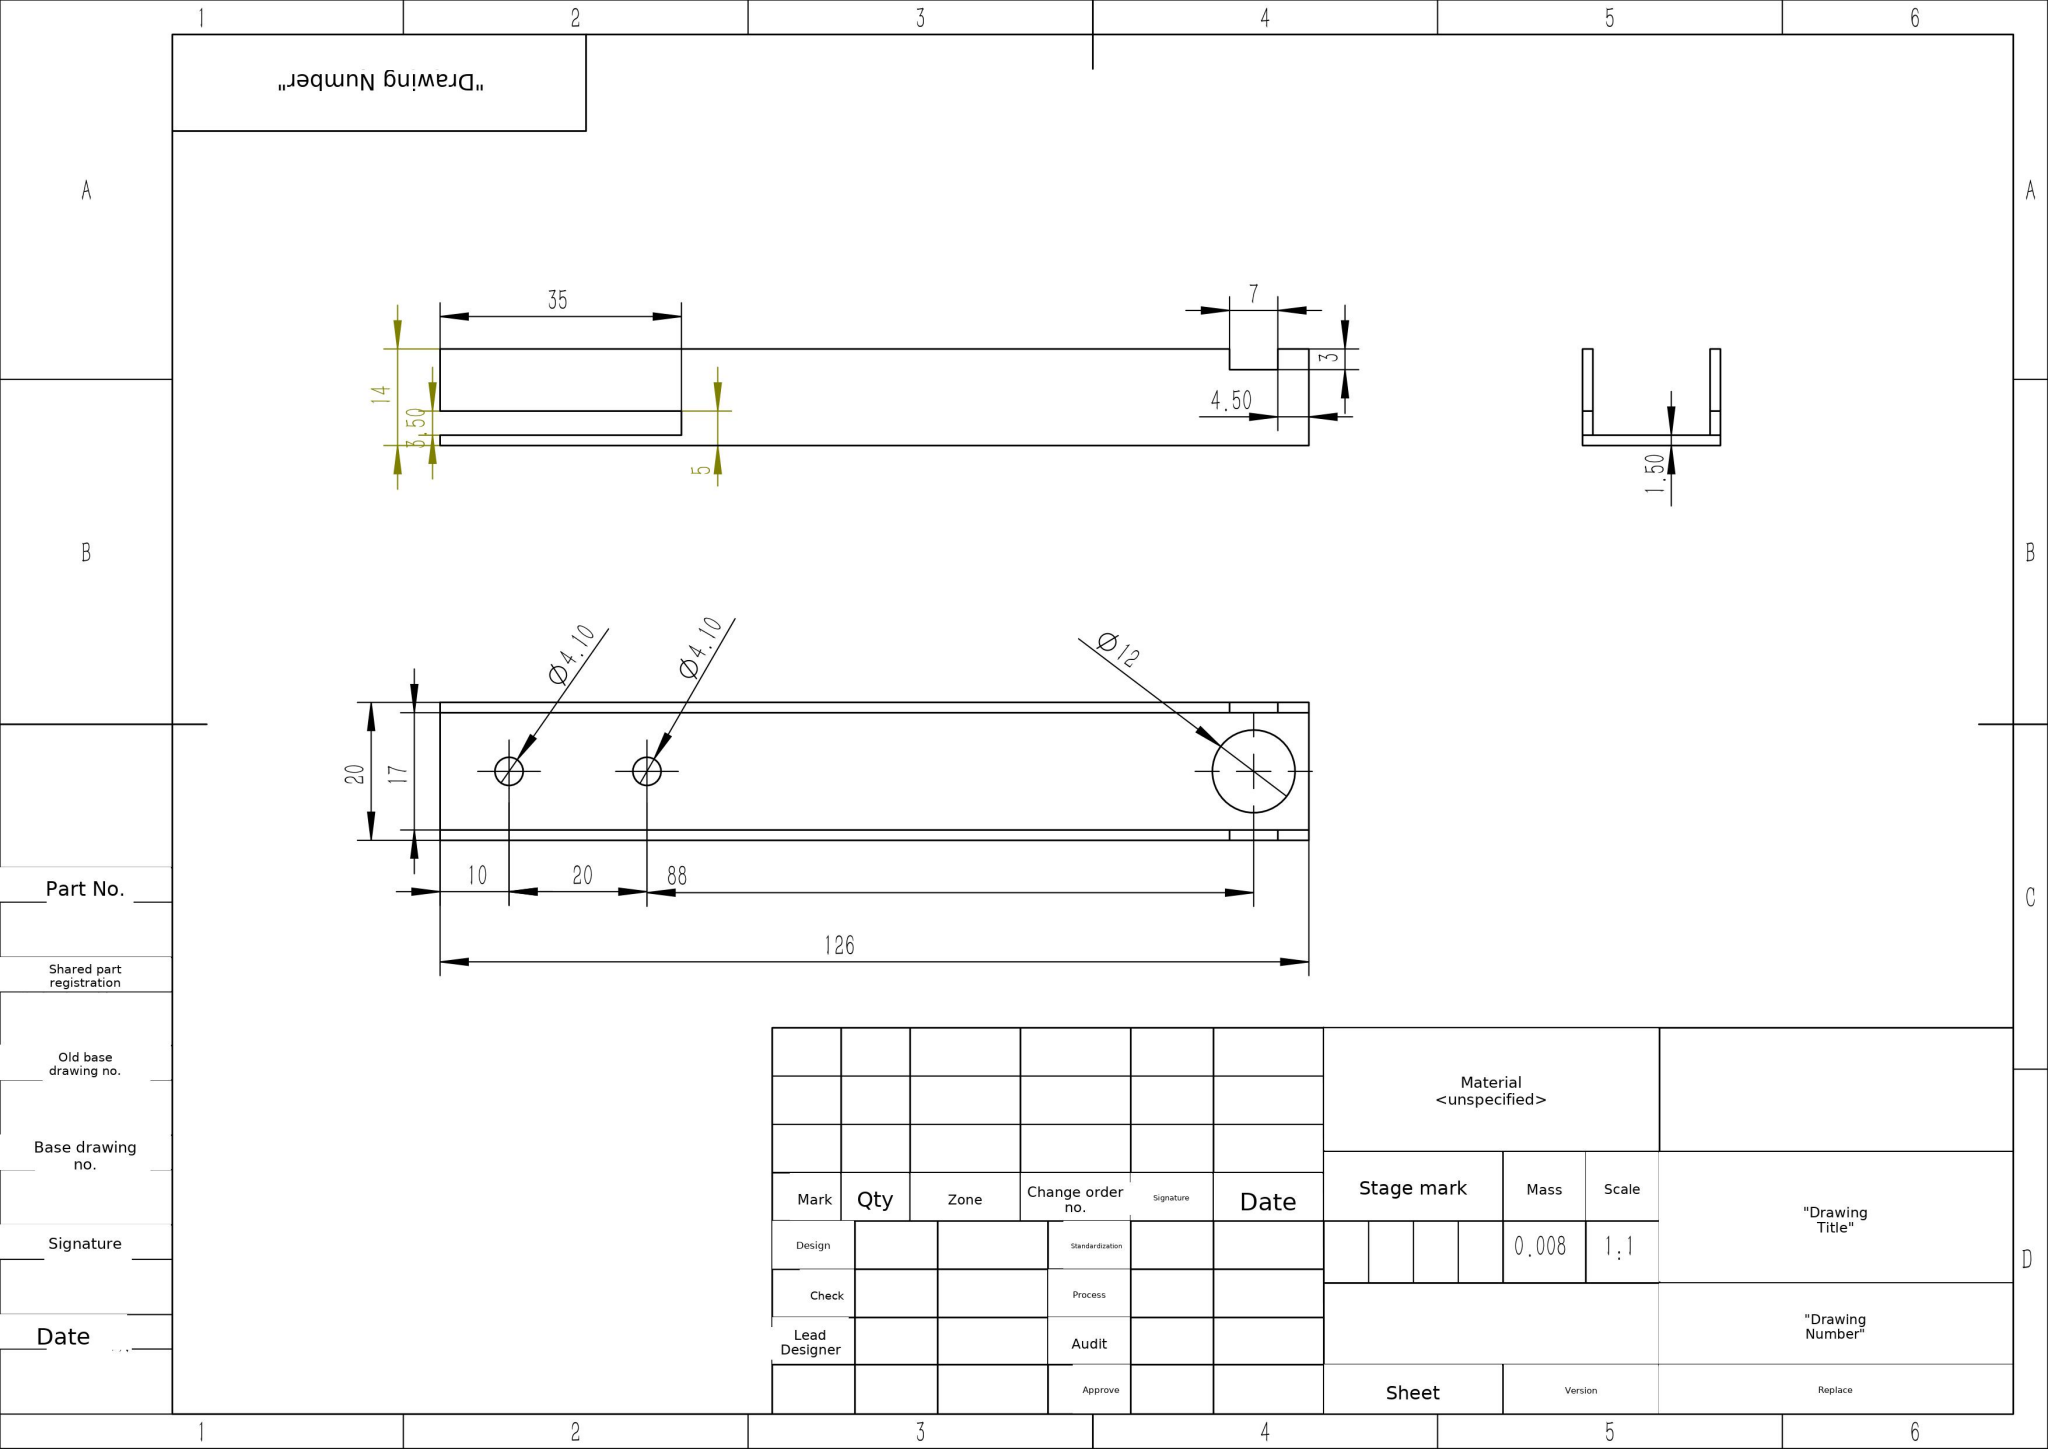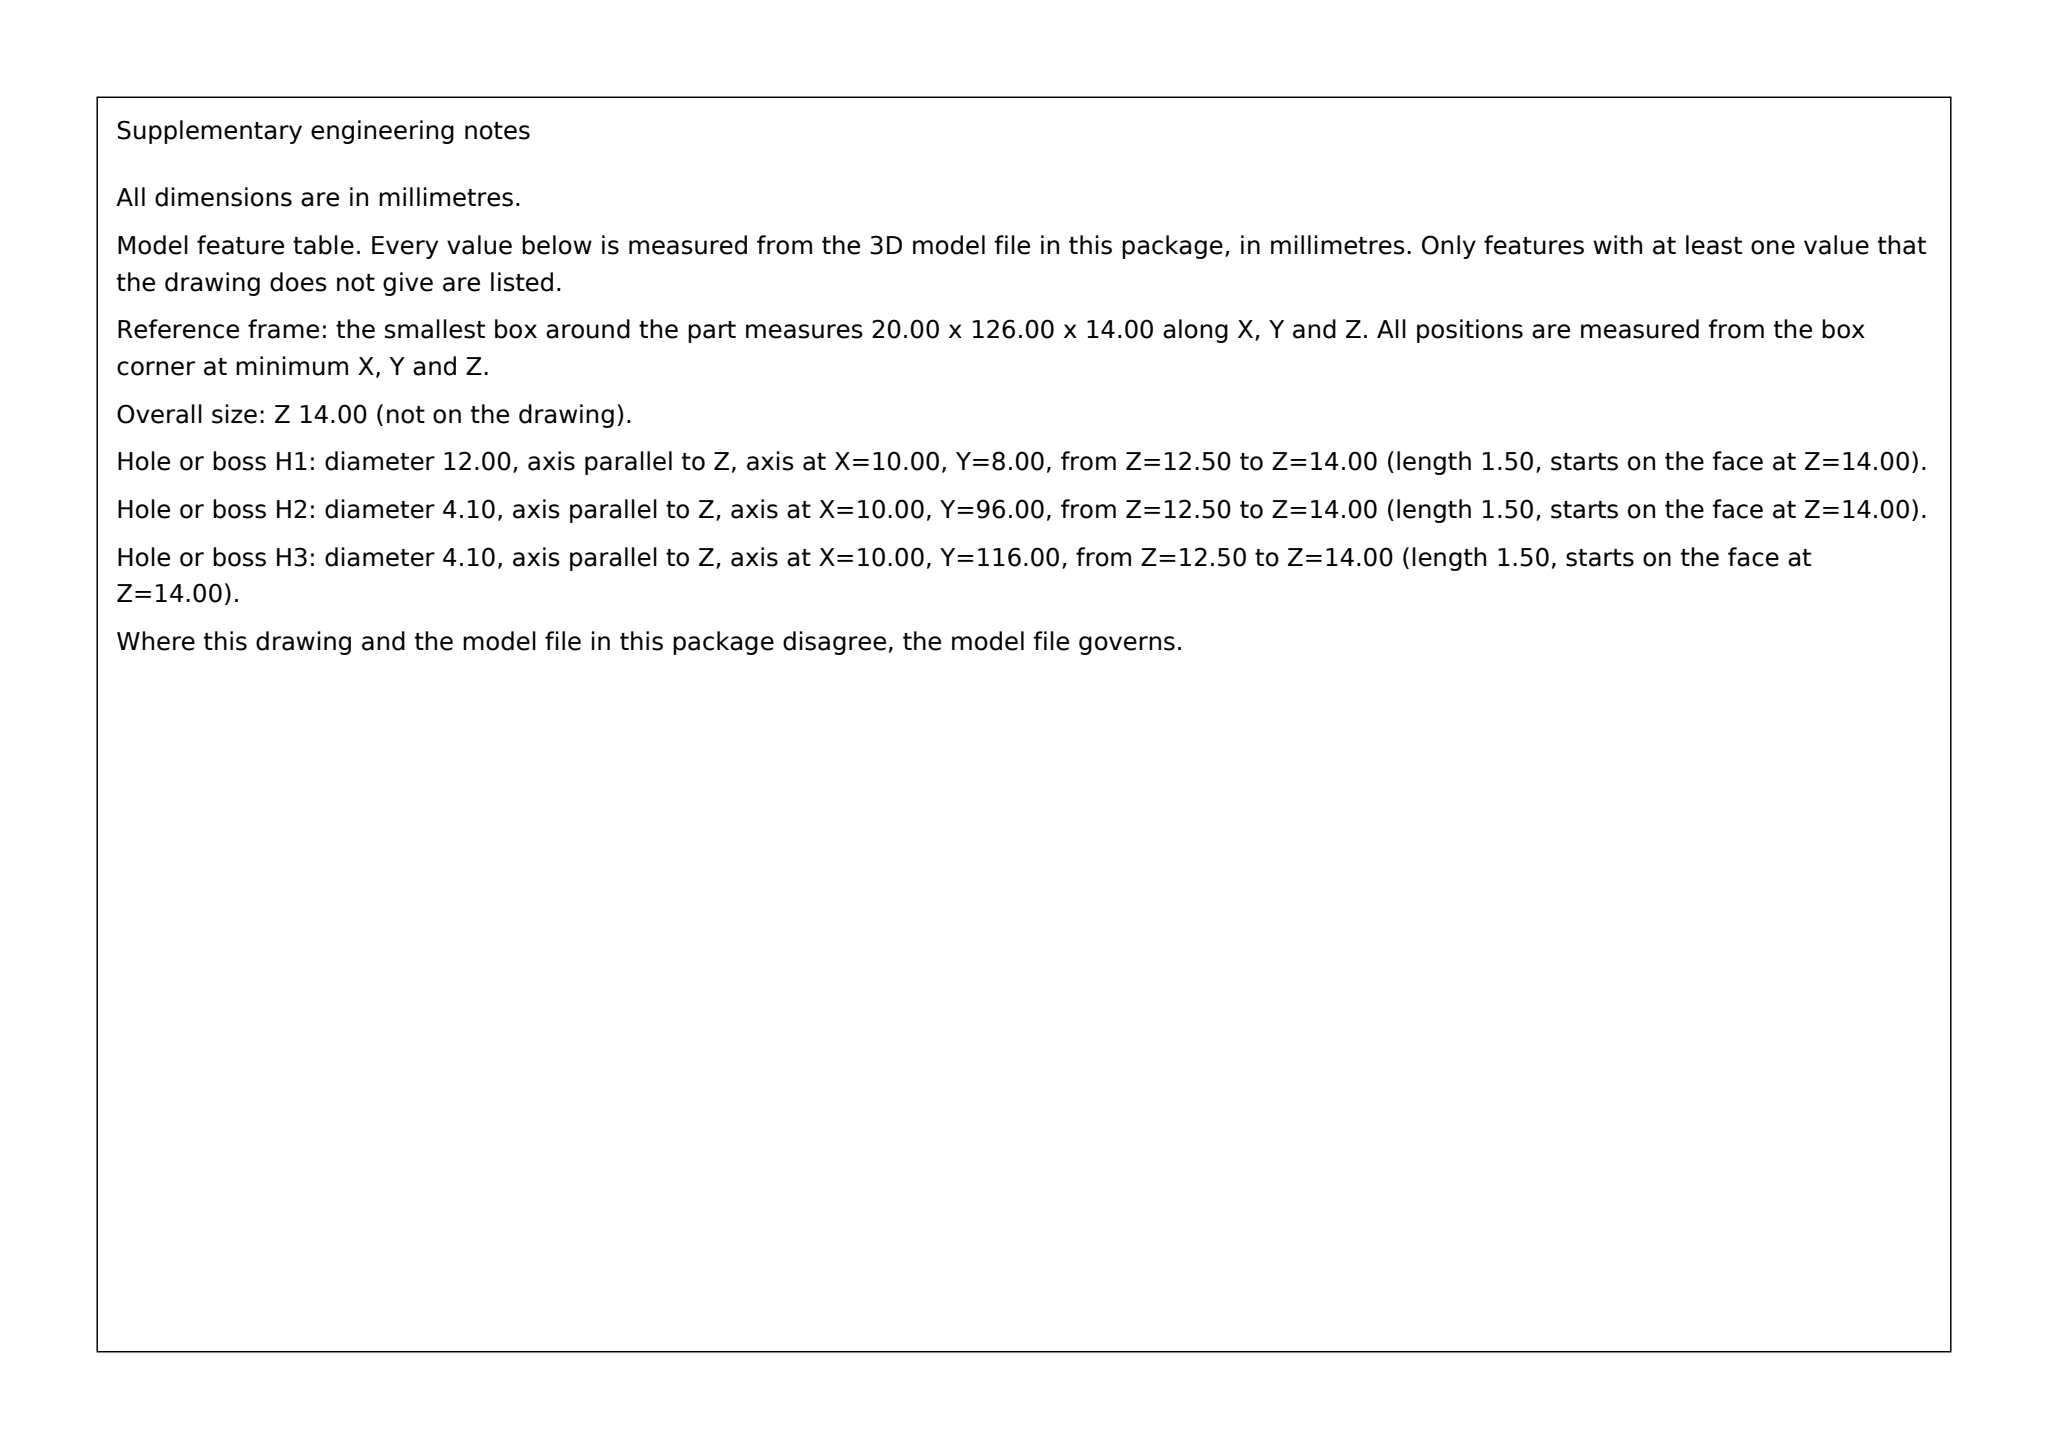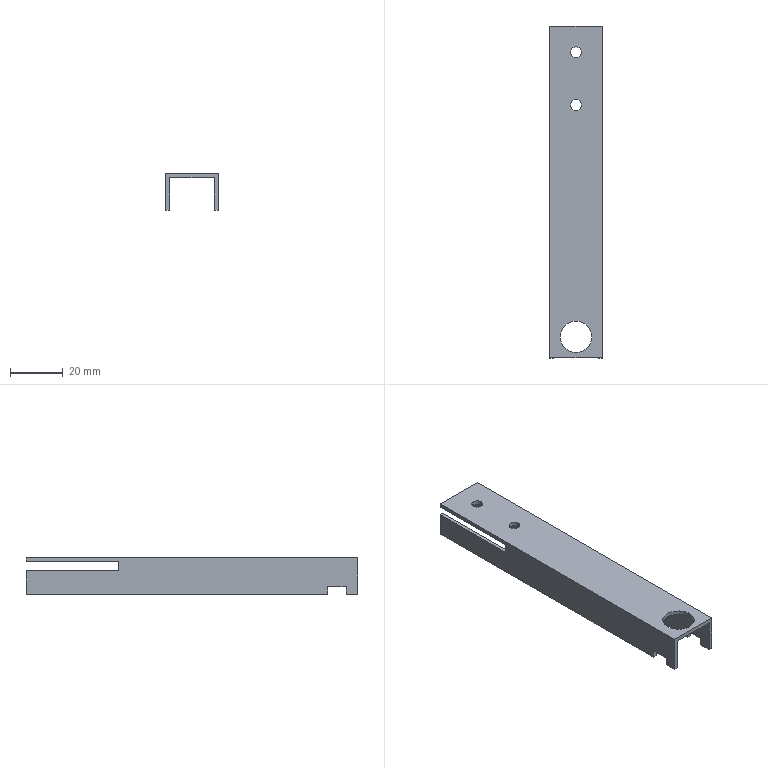Part | SolidWorks | mm | 1 solid | 30 faces | box 20 x 126 x 14 mm | volume 7865 mm3 | plane 24 | cylinder 6 | commonest cylinder face diameters 4.1 x4 12 x2
build123d program:
from build123d import *

# Parameters (mm, degrees)
BOSS_EXTRUDE1_DEPTH = 126
SKETCH2_W           = 3.5
SKETCH2_H           = 35
CUT_EXTRUDE1_DEPTH  = 129.343
SKETCH3_R           = 2.05
SKETCH3_R_2         = 6
CUT_EXTRUDE2_DEPTH  = 129.188
SKETCH4_W           = 3
SKETCH4_H           = 7
CUT_EXTRUDE3_DEPTH  = 129.343


with BuildPart() as part:
    # Sketch1 → Boss-Extrude1 (new body)
    with BuildSketch(Plane(origin=(0, 0, 0), x_dir=(1, 0, 0), z_dir=(0, 1, 0))):
        Polygon((-20, 14), (-20, 1.5), (-20, 0), (-18.5, 0), (-1.5, 0), (0, 0), (0, 1.5), (0, 14), (-1.5, 14), (-1.5, 1.5), (-18.5, 1.5), (-18.5, 14), align=None)
    extrude(amount=BOSS_EXTRUDE1_DEPTH)

    # Sketch2 → Cut-Extrude1 (cut, through all)
    with BuildSketch(Plane(origin=(0, 0, 0), x_dir=(0, 0, -1), z_dir=(1, 0, 0))):
        with Locations((3.25, 108.5)):
            Rectangle(SKETCH2_W, SKETCH2_H)
    extrude(amount=-CUT_EXTRUDE1_DEPTH, mode=Mode.SUBTRACT)

    # Sketch3 → Cut-Extrude2 (cut, through all)
    with BuildSketch(Plane(origin=(0, 0, -1.5), x_dir=(-1, 0, 0), z_dir=(0, 0, -1))):
        with Locations((10, 116)):
            Circle(SKETCH3_R)
        with Locations((10, 96)):
            Circle(SKETCH3_R)
        with Locations((10, 8)):
            Circle(SKETCH3_R_2)
    extrude(amount=-CUT_EXTRUDE2_DEPTH, mode=Mode.SUBTRACT)

    # Sketch4 → Cut-Extrude3 (cut, through all)
    with BuildSketch(Plane(origin=(0, 0, 0), x_dir=(0, 0, -1), z_dir=(1, 0, 0))):
        with Locations((12.5, 8)):
            Rectangle(SKETCH4_W, SKETCH4_H)
    extrude(amount=-CUT_EXTRUDE3_DEPTH, mode=Mode.SUBTRACT)


solid = part.part